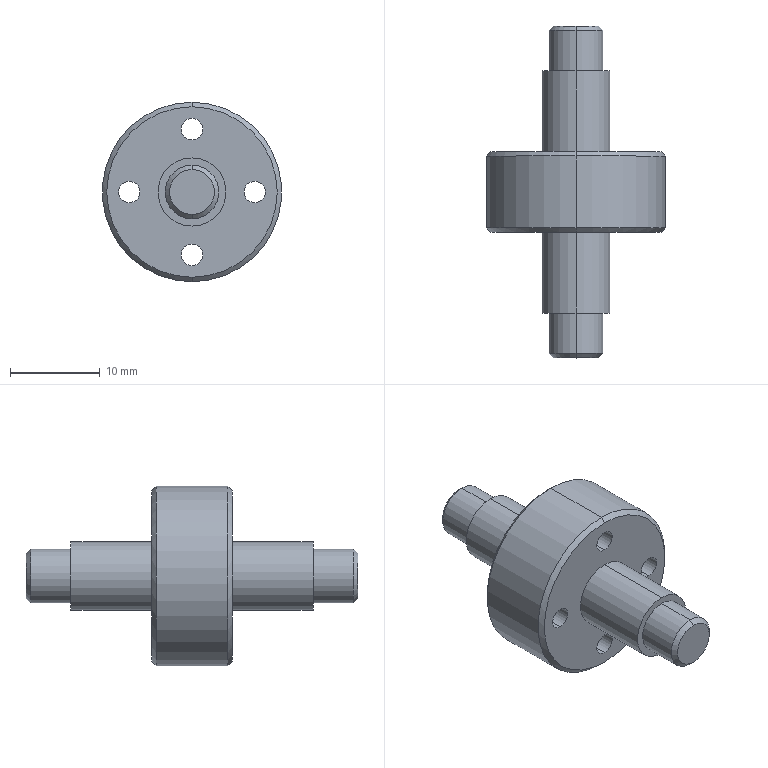Component | SolidWorks | FrontWheelAxis-1 | 1 solid | 32 faces | box 20 x 37 x 20 mm | volume 3744 mm3 | cylinder 18 | cone 8 | plane 6 | commonest cylinder face diameters 2.4 x8 6 x4 7.6 x4 20 x2 | material 6061 Alloy
build123d program:
from build123d import *

# Parameters (mm, degrees)
SKETCH1_R           = 10
SKETCH1_R_2         = 1.2
BOSS_EXTRUDE1_DEPTH = 9
SKETCH2_R           = 3.8
BOSS_EXTRUDE2_DEPTH = 9
SKETCH3_R           = 3
BOSS_EXTRUDE3_DEPTH = 5
BOSS_EXTRUDE4_START = 9
SKETCH4_R           = 3.8
BOSS_EXTRUDE4_DEPTH = 9
BOSS_EXTRUDE5_START = 5
SKETCH5_R           = 3
BOSS_EXTRUDE5_DEPTH = 5
CHAMFER1_SIZE       = 0.5


with BuildPart() as part:
    # Sketch1 → Boss-Extrude1 (new body)
    with BuildSketch(Plane(origin=(0, 0, 0), x_dir=(1, 0, 0), z_dir=(0, 1, 0))):
        with Locations(Location((0, 0, 0), (0, 0, 270))):
            Circle(SKETCH1_R)
        with Locations(Location((7, 0, 0), (0, 0, 270))):
            Circle(SKETCH1_R_2, mode=Mode.SUBTRACT)
        with Locations(Location((0, -7, 0), (0, 0, 270))):
            Circle(SKETCH1_R_2, mode=Mode.SUBTRACT)
        with Locations(Location((-7, 0, 0), (0, 0, 270))):
            Circle(SKETCH1_R_2, mode=Mode.SUBTRACT)
        with Locations(Location((0, 7, 0), (0, 0, 270))):
            Circle(SKETCH1_R_2, mode=Mode.SUBTRACT)
    extrude(amount=BOSS_EXTRUDE1_DEPTH)

    # Sketch2 → Boss-Extrude2 (add)
    with BuildSketch(Plane(origin=(0, 9, 0), x_dir=(1, 0, 0), z_dir=(0, 1, 0))):
        with Locations(Location((0, 0, 0), (0, 0, 270))):
            Circle(SKETCH2_R)
    extrude(amount=BOSS_EXTRUDE2_DEPTH)

    # Sketch3 → Boss-Extrude3 (add)
    with BuildSketch(Plane(origin=(0, 18, 0), x_dir=(1, 0, 0), z_dir=(0, 1, 0))):
        with Locations(Location((0, 0, 0), (0, 0, 270))):
            Circle(SKETCH3_R)
    extrude(amount=BOSS_EXTRUDE3_DEPTH)

    # Sketch4 → Boss-Extrude4 (add)
    with BuildSketch(Plane.XZ.offset(BOSS_EXTRUDE4_START)):
        with Locations(Location((0, 0, 0), (0, 0, 90))):
            Circle(SKETCH4_R)
    extrude(amount=-BOSS_EXTRUDE4_DEPTH)

    # Sketch5 → Boss-Extrude5 (add)
    with BuildSketch(Plane.XZ.offset(9).offset(BOSS_EXTRUDE5_START)):
        with Locations(Location((0, 0, 0), (0, 0, 90))):
            Circle(SKETCH5_R)
    extrude(amount=-BOSS_EXTRUDE5_DEPTH)

    # Chamfer1
    chamfer1_edges = [part.edges().sort_by_distance(p)[0] for p in [
        (0, 0, -10),
        (0, 23, -3),
        (0, -14, -3),
        (0, 9, -10),
    ]]
    chamfer(chamfer1_edges, length=CHAMFER1_SIZE)


solid = part.part

# Placed as in the assembly
solid = solid.moved(Location((0.3183, -0.6003, 37), (0, 0, 0)))
STEP:
#1=CARTESIAN_POINT('',(0.01253,-0.5748,1.358));
#2=VERTEX_POINT('',#1);
#3=CARTESIAN_POINT('',(0.01253,-0.5748,1.555));
#4=VERTEX_POINT('',#3);
#5=CARTESIAN_POINT('',(0.01253,-0.5748,1.457));
#6=DIRECTION('',(0.,-1.,0.));
#7=DIRECTION('',(0.,0.,-1.));
#8=AXIS2_PLACEMENT_3D('',#5,#6,#7);
#9=CIRCLE('',#8,0.09843);
#10=EDGE_CURVE('',#2,#4,#9,.T.);
#11=ORIENTED_EDGE('',*,*,#10,.F.);
#12=CARTESIAN_POINT('',(0.01253,-0.5551,1.339));
#13=VERTEX_POINT('',#12);
#14=CARTESIAN_POINT('',(0.01253,-0.5748,1.358));
#15=DIRECTION('',(0.,0.7071,-0.7071));
#16=VECTOR('',#15,39.37);
#17=LINE('',#14,#16);
#18=EDGE_CURVE('',#2,#13,#17,.T.);
#19=ORIENTED_EDGE('',*,*,#18,.T.);
#20=CARTESIAN_POINT('',(0.01253,-0.5551,1.575));
#21=VERTEX_POINT('',#20);
#22=CARTESIAN_POINT('',(0.01253,-0.5551,1.457));
#23=DIRECTION('',(0.,1.,0.));
#24=DIRECTION('',(0.,0.,-1.));
#25=AXIS2_PLACEMENT_3D('',#22,#23,#24);
#26=CIRCLE('',#25,0.1181);
#27=EDGE_CURVE('',#21,#13,#26,.T.);
#28=ORIENTED_EDGE('',*,*,#27,.F.);
#29=CARTESIAN_POINT('',(0.01253,-0.5748,1.555));
#30=DIRECTION('',(0.,0.7071,0.7071));
#31=VECTOR('',#30,39.37);
#32=LINE('',#29,#31);
#33=EDGE_CURVE('',#4,#21,#32,.T.);
#34=ORIENTED_EDGE('',*,*,#33,.F.);
#35=EDGE_LOOP('',(#11,#19,#28,#34));
#36=FACE_OUTER_BOUND('',#35,.T.);
#37=CARTESIAN_POINT('',(0.01253,-0.5748,1.457));
#38=DIRECTION('',(0.,1.,0.));
#39=DIRECTION('',(0.,0.,1.));
#40=AXIS2_PLACEMENT_3D('',#37,#38,#39);
#41=CONICAL_SURFACE('',#40,0.09843,0.7854);
#42=ADVANCED_FACE('',(#36),#41,.T.);
#43=CARTESIAN_POINT('',(0.01253,0.8819,1.555));
#44=VERTEX_POINT('',#43);
#45=CARTESIAN_POINT('',(0.01253,0.8819,1.358));
#46=VERTEX_POINT('',#45);
#47=CARTESIAN_POINT('',(0.01253,0.8819,1.457));
#48=DIRECTION('',(0.,1.,0.));
#49=DIRECTION('',(0.,0.,1.));
#50=AXIS2_PLACEMENT_3D('',#47,#48,#49);
#51=CIRCLE('',#50,0.09843);
#52=EDGE_CURVE('',#44,#46,#51,.T.);
#53=ORIENTED_EDGE('',*,*,#52,.F.);
#54=CARTESIAN_POINT('',(0.01253,0.8622,1.575));
#55=VERTEX_POINT('',#54);
#56=CARTESIAN_POINT('',(0.01253,0.8819,1.555));
#57=DIRECTION('',(0.,-0.7071,0.7071));
#58=VECTOR('',#57,39.37);
#59=LINE('',#56,#58);
#60=EDGE_CURVE('',#44,#55,#59,.T.);
#61=ORIENTED_EDGE('',*,*,#60,.T.);
#62=CARTESIAN_POINT('',(0.01253,0.8622,1.339));
#63=VERTEX_POINT('',#62);
#64=CARTESIAN_POINT('',(0.01253,0.8622,1.457));
#65=DIRECTION('',(0.,-1.,0.));
#66=DIRECTION('',(0.,0.,1.));
#67=AXIS2_PLACEMENT_3D('',#64,#65,#66);
#68=CIRCLE('',#67,0.1181);
#69=EDGE_CURVE('',#63,#55,#68,.T.);
#70=ORIENTED_EDGE('',*,*,#69,.F.);
#71=CARTESIAN_POINT('',(0.01253,0.8819,1.358));
#72=DIRECTION('',(0.,-0.7071,-0.7071));
#73=VECTOR('',#72,39.37);
#74=LINE('',#71,#73);
#75=EDGE_CURVE('',#46,#63,#74,.T.);
#76=ORIENTED_EDGE('',*,*,#75,.F.);
#77=EDGE_LOOP('',(#53,#61,#70,#76));
#78=FACE_OUTER_BOUND('',#77,.T.);
#79=CARTESIAN_POINT('',(0.01253,0.8819,1.457));
#80=DIRECTION('',(0.,-1.,0.));
#81=DIRECTION('',(0.,0.,-1.));
#82=AXIS2_PLACEMENT_3D('',#79,#80,#81);
#83=CONICAL_SURFACE('',#82,0.09843,0.7854);
#84=ADVANCED_FACE('',(#78),#83,.T.);
#85=CARTESIAN_POINT('',(0.01253,-0.02363,1.083));
#86=VERTEX_POINT('',#85);
#87=CARTESIAN_POINT('',(0.01253,-0.02363,1.831));
#88=VERTEX_POINT('',#87);
#89=CARTESIAN_POINT('',(0.01253,-0.02363,1.457));
#90=DIRECTION('',(0.,-1.,0.));
#91=DIRECTION('',(0.,0.,1.));
#92=AXIS2_PLACEMENT_3D('',#89,#90,#91);
#93=CIRCLE('',#92,0.374);
#94=EDGE_CURVE('',#86,#88,#93,.T.);
#95=ORIENTED_EDGE('',*,*,#94,.F.);
#96=CARTESIAN_POINT('',(0.01253,-0.003948,1.063));
#97=VERTEX_POINT('',#96);
#98=CARTESIAN_POINT('',(0.01253,-0.003948,1.063));
#99=DIRECTION('',(0.,0.7071,-0.7071));
#100=VECTOR('',#99,39.37);
#101=LINE('',#98,#100);
#102=EDGE_CURVE('',#86,#97,#101,.T.);
#103=ORIENTED_EDGE('',*,*,#102,.T.);
#104=CARTESIAN_POINT('',(0.01253,-0.003948,1.85));
#105=VERTEX_POINT('',#104);
#106=CARTESIAN_POINT('',(0.01253,-0.003948,1.457));
#107=DIRECTION('',(0.,1.,0.));
#108=DIRECTION('',(0.,0.,1.));
#109=AXIS2_PLACEMENT_3D('',#106,#107,#108);
#110=CIRCLE('',#109,0.3937);
#111=EDGE_CURVE('',#105,#97,#110,.T.);
#112=ORIENTED_EDGE('',*,*,#111,.F.);
#113=CARTESIAN_POINT('',(0.01253,-0.003948,1.85));
#114=DIRECTION('',(0.,0.7071,0.7071));
#115=VECTOR('',#114,39.37);
#116=LINE('',#113,#115);
#117=EDGE_CURVE('',#88,#105,#116,.T.);
#118=ORIENTED_EDGE('',*,*,#117,.F.);
#119=EDGE_LOOP('',(#95,#103,#112,#118));
#120=FACE_OUTER_BOUND('',#119,.T.);
#121=CARTESIAN_POINT('',(0.01253,-0.003948,1.457));
#122=DIRECTION('',(0.,1.,0.));
#123=DIRECTION('',(0.,0.,1.));
#124=AXIS2_PLACEMENT_3D('',#121,#122,#123);
#125=CONICAL_SURFACE('',#124,0.3937,0.7854);
#126=ADVANCED_FACE('',(#120),#125,.T.);
#127=CARTESIAN_POINT('',(0.01253,0.3307,1.831));
#128=VERTEX_POINT('',#127);
#129=CARTESIAN_POINT('',(0.01253,0.3307,1.083));
#130=VERTEX_POINT('',#129);
#131=CARTESIAN_POINT('',(0.01253,0.3307,1.457));
#132=DIRECTION('',(0.,1.,0.));
#133=DIRECTION('',(0.,0.,1.));
#134=AXIS2_PLACEMENT_3D('',#131,#132,#133);
#135=CIRCLE('',#134,0.374);
#136=EDGE_CURVE('',#128,#130,#135,.T.);
#137=ORIENTED_EDGE('',*,*,#136,.F.);
#138=CARTESIAN_POINT('',(0.01253,0.311,1.85));
#139=VERTEX_POINT('',#138);
#140=CARTESIAN_POINT('',(0.01253,0.3307,1.831));
#141=DIRECTION('',(0.,-0.7071,0.7071));
#142=VECTOR('',#141,39.37);
#143=LINE('',#140,#142);
#144=EDGE_CURVE('',#128,#139,#143,.T.);
#145=ORIENTED_EDGE('',*,*,#144,.T.);
#146=CARTESIAN_POINT('',(0.01253,0.311,1.063));
#147=VERTEX_POINT('',#146);
#148=CARTESIAN_POINT('',(0.01253,0.311,1.457));
#149=DIRECTION('',(0.,-1.,0.));
#150=DIRECTION('',(0.,0.,1.));
#151=AXIS2_PLACEMENT_3D('',#148,#149,#150);
#152=CIRCLE('',#151,0.3937);
#153=EDGE_CURVE('',#147,#139,#152,.T.);
#154=ORIENTED_EDGE('',*,*,#153,.F.);
#155=CARTESIAN_POINT('',(0.01253,0.3307,1.083));
#156=DIRECTION('',(0.,-0.7071,-0.7071));
#157=VECTOR('',#156,39.37);
#158=LINE('',#155,#157);
#159=EDGE_CURVE('',#130,#147,#158,.T.);
#160=ORIENTED_EDGE('',*,*,#159,.F.);
#161=EDGE_LOOP('',(#137,#145,#154,#160));
#162=FACE_OUTER_BOUND('',#161,.T.);
#163=CARTESIAN_POINT('',(0.01253,0.3307,1.457));
#164=DIRECTION('',(0.,-1.,0.));
#165=DIRECTION('',(0.,0.,-1.));
#166=AXIS2_PLACEMENT_3D('',#163,#164,#165);
#167=CONICAL_SURFACE('',#166,0.374,0.7854);
#168=ADVANCED_FACE('',(#162),#167,.T.);
#169=ORIENTED_EDGE('',*,*,#27,.T.);
#170=CARTESIAN_POINT('',(0.01253,-0.378,1.339));
#171=VERTEX_POINT('',#170);
#172=CARTESIAN_POINT('',(0.01253,-0.5748,1.339));
#173=DIRECTION('',(0.,1.,0.));
#174=VECTOR('',#173,39.37);
#175=LINE('',#172,#174);
#176=EDGE_CURVE('',#13,#171,#175,.T.);
#177=ORIENTED_EDGE('',*,*,#176,.T.);
#178=CARTESIAN_POINT('',(0.01253,-0.378,1.575));
#179=VERTEX_POINT('',#178);
#180=CARTESIAN_POINT('',(0.01253,-0.378,1.457));
#181=DIRECTION('',(0.,-1.,0.));
#182=DIRECTION('',(0.,0.,-1.));
#183=AXIS2_PLACEMENT_3D('',#180,#181,#182);
#184=CIRCLE('',#183,0.1181);
#185=EDGE_CURVE('',#171,#179,#184,.T.);
#186=ORIENTED_EDGE('',*,*,#185,.T.);
#187=CARTESIAN_POINT('',(0.01253,-0.5748,1.575));
#188=DIRECTION('',(0.,1.,0.));
#189=VECTOR('',#188,39.37);
#190=LINE('',#187,#189);
#191=EDGE_CURVE('',#21,#179,#190,.T.);
#192=ORIENTED_EDGE('',*,*,#191,.F.);
#193=EDGE_LOOP('',(#169,#177,#186,#192));
#194=FACE_OUTER_BOUND('',#193,.T.);
#195=CARTESIAN_POINT('',(0.01253,-0.5748,1.457));
#196=DIRECTION('',(0.,1.,0.));
#197=DIRECTION('',(0.,0.,1.));
#198=AXIS2_PLACEMENT_3D('',#195,#196,#197);
#199=CYLINDRICAL_SURFACE('',#198,0.1181);
#200=ADVANCED_FACE('',(#194),#199,.T.);
#201=CARTESIAN_POINT('',(0.01253,-0.378,1.307));
#202=VERTEX_POINT('',#201);
#203=CARTESIAN_POINT('',(0.01253,-0.378,1.606));
#204=VERTEX_POINT('',#203);
#205=CARTESIAN_POINT('',(0.01253,-0.378,1.457));
#206=DIRECTION('',(0.,-1.,0.));
#207=DIRECTION('',(0.,0.,-1.));
#208=AXIS2_PLACEMENT_3D('',#205,#206,#207);
#209=CIRCLE('',#208,0.1496);
#210=EDGE_CURVE('',#202,#204,#209,.T.);
#211=ORIENTED_EDGE('',*,*,#210,.F.);
#212=CARTESIAN_POINT('',(0.01253,-0.02363,1.307));
#213=VERTEX_POINT('',#212);
#214=CARTESIAN_POINT('',(0.01253,-0.378,1.307));
#215=DIRECTION('',(0.,1.,0.));
#216=VECTOR('',#215,39.37);
#217=LINE('',#214,#216);
#218=EDGE_CURVE('',#202,#213,#217,.T.);
#219=ORIENTED_EDGE('',*,*,#218,.T.);
#220=CARTESIAN_POINT('',(0.01253,-0.02363,1.606));
#221=VERTEX_POINT('',#220);
#222=CARTESIAN_POINT('',(0.01253,-0.02363,1.457));
#223=DIRECTION('',(0.,-1.,0.));
#224=DIRECTION('',(0.,0.,1.));
#225=AXIS2_PLACEMENT_3D('',#222,#223,#224);
#226=CIRCLE('',#225,0.1496);
#227=EDGE_CURVE('',#213,#221,#226,.T.);
#228=ORIENTED_EDGE('',*,*,#227,.T.);
#229=CARTESIAN_POINT('',(0.01253,-0.378,1.606));
#230=DIRECTION('',(0.,1.,0.));
#231=VECTOR('',#230,39.37);
#232=LINE('',#229,#231);
#233=EDGE_CURVE('',#204,#221,#232,.T.);
#234=ORIENTED_EDGE('',*,*,#233,.F.);
#235=EDGE_LOOP('',(#211,#219,#228,#234));
#236=FACE_OUTER_BOUND('',#235,.T.);
#237=CARTESIAN_POINT('',(0.01253,-0.378,1.457));
#238=DIRECTION('',(0.,1.,0.));
#239=DIRECTION('',(0.,0.,1.));
#240=AXIS2_PLACEMENT_3D('',#237,#238,#239);
#241=CYLINDRICAL_SURFACE('',#240,0.1496);
#242=ADVANCED_FACE('',(#236),#241,.T.);
#243=ORIENTED_EDGE('',*,*,#69,.T.);
#244=CARTESIAN_POINT('',(0.01253,0.685,1.575));
#245=VERTEX_POINT('',#244);
#246=CARTESIAN_POINT('',(0.01253,0.8819,1.575));
#247=DIRECTION('',(0.,-1.,0.));
#248=VECTOR('',#247,39.37);
#249=LINE('',#246,#248);
#250=EDGE_CURVE('',#55,#245,#249,.T.);
#251=ORIENTED_EDGE('',*,*,#250,.T.);
#252=CARTESIAN_POINT('',(0.01253,0.685,1.339));
#253=VERTEX_POINT('',#252);
#254=CARTESIAN_POINT('',(0.01253,0.685,1.457));
#255=DIRECTION('',(0.,1.,0.));
#256=DIRECTION('',(0.,0.,1.));
#257=AXIS2_PLACEMENT_3D('',#254,#255,#256);
#258=CIRCLE('',#257,0.1181);
#259=EDGE_CURVE('',#245,#253,#258,.T.);
#260=ORIENTED_EDGE('',*,*,#259,.T.);
#261=CARTESIAN_POINT('',(0.01253,0.8819,1.339));
#262=DIRECTION('',(0.,-1.,0.));
#263=VECTOR('',#262,39.37);
#264=LINE('',#261,#263);
#265=EDGE_CURVE('',#63,#253,#264,.T.);
#266=ORIENTED_EDGE('',*,*,#265,.F.);
#267=EDGE_LOOP('',(#243,#251,#260,#266));
#268=FACE_OUTER_BOUND('',#267,.T.);
#269=CARTESIAN_POINT('',(0.01253,0.8819,1.457));
#270=DIRECTION('',(0.,-1.,0.));
#271=DIRECTION('',(0.,0.,-1.));
#272=AXIS2_PLACEMENT_3D('',#269,#270,#271);
#273=CYLINDRICAL_SURFACE('',#272,0.1181);
#274=ADVANCED_FACE('',(#268),#273,.T.);
#275=CARTESIAN_POINT('',(0.01253,0.685,1.606));
#276=VERTEX_POINT('',#275);
#277=CARTESIAN_POINT('',(0.01253,0.685,1.307));
#278=VERTEX_POINT('',#277);
#279=CARTESIAN_POINT('',(0.01253,0.685,1.457));
#280=DIRECTION('',(0.,1.,0.));
#281=DIRECTION('',(0.,0.,1.));
#282=AXIS2_PLACEMENT_3D('',#279,#280,#281);
#283=CIRCLE('',#282,0.1496);
#284=EDGE_CURVE('',#276,#278,#283,.T.);
#285=ORIENTED_EDGE('',*,*,#284,.F.);
#286=CARTESIAN_POINT('',(0.01253,0.3307,1.606));
#287=VERTEX_POINT('',#286);
#288=CARTESIAN_POINT('',(0.01253,0.685,1.606));
#289=DIRECTION('',(0.,-1.,0.));
#290=VECTOR('',#289,39.37);
#291=LINE('',#288,#290);
#292=EDGE_CURVE('',#276,#287,#291,.T.);
#293=ORIENTED_EDGE('',*,*,#292,.T.);
#294=CARTESIAN_POINT('',(0.01253,0.3307,1.307));
#295=VERTEX_POINT('',#294);
#296=CARTESIAN_POINT('',(0.01253,0.3307,1.457));
#297=DIRECTION('',(0.,1.,0.));
#298=DIRECTION('',(0.,0.,1.));
#299=AXIS2_PLACEMENT_3D('',#296,#297,#298);
#300=CIRCLE('',#299,0.1496);
#301=EDGE_CURVE('',#287,#295,#300,.T.);
#302=ORIENTED_EDGE('',*,*,#301,.T.);
#303=CARTESIAN_POINT('',(0.01253,0.685,1.307));
#304=DIRECTION('',(0.,-1.,0.));
#305=VECTOR('',#304,39.37);
#306=LINE('',#303,#305);
#307=EDGE_CURVE('',#278,#295,#306,.T.);
#308=ORIENTED_EDGE('',*,*,#307,.F.);
#309=EDGE_LOOP('',(#285,#293,#302,#308));
#310=FACE_OUTER_BOUND('',#309,.T.);
#311=CARTESIAN_POINT('',(0.01253,0.685,1.457));
#312=DIRECTION('',(0.,-1.,0.));
#313=DIRECTION('',(0.,0.,-1.));
#314=AXIS2_PLACEMENT_3D('',#311,#312,#313);
#315=CYLINDRICAL_SURFACE('',#314,0.1496);
#316=ADVANCED_FACE('',(#310),#315,.T.);
#317=CARTESIAN_POINT('',(0.01253,0.3307,1.134));
#318=VERTEX_POINT('',#317);
#319=CARTESIAN_POINT('',(0.01253,0.3307,1.228));
#320=VERTEX_POINT('',#319);
#321=CARTESIAN_POINT('',(0.01253,0.3307,1.181));
#322=DIRECTION('',(0.,1.,0.));
#323=DIRECTION('',(0.,0.,1.));
#324=AXIS2_PLACEMENT_3D('',#321,#322,#323);
#325=CIRCLE('',#324,0.04724);
#326=EDGE_CURVE('',#318,#320,#325,.T.);
#327=ORIENTED_EDGE('',*,*,#326,.T.);
#328=CARTESIAN_POINT('',(0.01253,-0.02363,1.228));
#329=VERTEX_POINT('',#328);
#330=CARTESIAN_POINT('',(0.01253,0.3307,1.228));
#331=DIRECTION('',(0.,-1.,0.));
#332=VECTOR('',#331,39.37);
#333=LINE('',#330,#332);
#334=EDGE_CURVE('',#320,#329,#333,.T.);
#335=ORIENTED_EDGE('',*,*,#334,.T.);
#336=CARTESIAN_POINT('',(0.01253,-0.02363,1.134));
#337=VERTEX_POINT('',#336);
#338=CARTESIAN_POINT('',(0.01253,-0.02363,1.181));
#339=DIRECTION('',(0.,1.,0.));
#340=DIRECTION('',(0.,0.,1.));
#341=AXIS2_PLACEMENT_3D('',#338,#339,#340);
#342=CIRCLE('',#341,0.04724);
#343=EDGE_CURVE('',#337,#329,#342,.T.);
#344=ORIENTED_EDGE('',*,*,#343,.F.);
#345=CARTESIAN_POINT('',(0.01253,0.3307,1.134));
#346=DIRECTION('',(0.,-1.,0.));
#347=VECTOR('',#346,39.37);
#348=LINE('',#345,#347);
#349=EDGE_CURVE('',#318,#337,#348,.T.);
#350=ORIENTED_EDGE('',*,*,#349,.F.);
#351=EDGE_LOOP('',(#327,#335,#344,#350));
#352=FACE_OUTER_BOUND('',#351,.T.);
#353=CARTESIAN_POINT('',(0.01253,0.3307,1.181));
#354=DIRECTION('',(0.,-1.,0.));
#355=DIRECTION('',(0.,0.,-1.));
#356=AXIS2_PLACEMENT_3D('',#353,#354,#355);
#357=CYLINDRICAL_SURFACE('',#356,0.04724);
#358=ADVANCED_FACE('',(#352),#357,.F.);
#359=CARTESIAN_POINT('',(-0.2631,0.3307,1.409));
#360=VERTEX_POINT('',#359);
#361=CARTESIAN_POINT('',(-0.2631,0.3307,1.504));
#362=VERTEX_POINT('',#361);
#363=CARTESIAN_POINT('',(-0.2631,0.3307,1.457));
#364=DIRECTION('',(0.,1.,0.));
#365=DIRECTION('',(0.,0.,1.));
#366=AXIS2_PLACEMENT_3D('',#363,#364,#365);
#367=CIRCLE('',#366,0.04724);
#368=EDGE_CURVE('',#360,#362,#367,.T.);
#369=ORIENTED_EDGE('',*,*,#368,.T.);
#370=CARTESIAN_POINT('',(-0.2631,-0.02363,1.504));
#371=VERTEX_POINT('',#370);
#372=CARTESIAN_POINT('',(-0.2631,0.3307,1.504));
#373=DIRECTION('',(0.,-1.,0.));
#374=VECTOR('',#373,39.37);
#375=LINE('',#372,#374);
#376=EDGE_CURVE('',#362,#371,#375,.T.);
#377=ORIENTED_EDGE('',*,*,#376,.T.);
#378=CARTESIAN_POINT('',(-0.2631,-0.02363,1.409));
#379=VERTEX_POINT('',#378);
#380=CARTESIAN_POINT('',(-0.2631,-0.02363,1.457));
#381=DIRECTION('',(0.,1.,0.));
#382=DIRECTION('',(0.,0.,1.));
#383=AXIS2_PLACEMENT_3D('',#380,#381,#382);
#384=CIRCLE('',#383,0.04724);
#385=EDGE_CURVE('',#379,#371,#384,.T.);
#386=ORIENTED_EDGE('',*,*,#385,.F.);
#387=CARTESIAN_POINT('',(-0.2631,0.3307,1.409));
#388=DIRECTION('',(0.,-1.,0.));
#389=VECTOR('',#388,39.37);
#390=LINE('',#387,#389);
#391=EDGE_CURVE('',#360,#379,#390,.T.);
#392=ORIENTED_EDGE('',*,*,#391,.F.);
#393=EDGE_LOOP('',(#369,#377,#386,#392));
#394=FACE_OUTER_BOUND('',#393,.T.);
#395=CARTESIAN_POINT('',(-0.2631,0.3307,1.457));
#396=DIRECTION('',(0.,-1.,0.));
#397=DIRECTION('',(0.,0.,-1.));
#398=AXIS2_PLACEMENT_3D('',#395,#396,#397);
#399=CYLINDRICAL_SURFACE('',#398,0.04724);
#400=ADVANCED_FACE('',(#394),#399,.F.);
#401=CARTESIAN_POINT('',(0.01253,0.3307,1.685));
#402=VERTEX_POINT('',#401);
#403=CARTESIAN_POINT('',(0.01253,0.3307,1.78));
#404=VERTEX_POINT('',#403);
#405=CARTESIAN_POINT('',(0.01253,0.3307,1.732));
#406=DIRECTION('',(0.,1.,0.));
#407=DIRECTION('',(0.,0.,1.));
#408=AXIS2_PLACEMENT_3D('',#405,#406,#407);
#409=CIRCLE('',#408,0.04724);
#410=EDGE_CURVE('',#402,#404,#409,.T.);
#411=ORIENTED_EDGE('',*,*,#410,.T.);
#412=CARTESIAN_POINT('',(0.01253,-0.02363,1.78));
#413=VERTEX_POINT('',#412);
#414=CARTESIAN_POINT('',(0.01253,0.3307,1.78));
#415=DIRECTION('',(0.,-1.,0.));
#416=VECTOR('',#415,39.37);
#417=LINE('',#414,#416);
#418=EDGE_CURVE('',#404,#413,#417,.T.);
#419=ORIENTED_EDGE('',*,*,#418,.T.);
#420=CARTESIAN_POINT('',(0.01253,-0.02363,1.685));
#421=VERTEX_POINT('',#420);
#422=CARTESIAN_POINT('',(0.01253,-0.02363,1.732));
#423=DIRECTION('',(0.,1.,0.));
#424=DIRECTION('',(0.,0.,1.));
#425=AXIS2_PLACEMENT_3D('',#422,#423,#424);
#426=CIRCLE('',#425,0.04724);
#427=EDGE_CURVE('',#421,#413,#426,.T.);
#428=ORIENTED_EDGE('',*,*,#427,.F.);
#429=CARTESIAN_POINT('',(0.01253,0.3307,1.685));
#430=DIRECTION('',(0.,-1.,0.));
#431=VECTOR('',#430,39.37);
#432=LINE('',#429,#431);
#433=EDGE_CURVE('',#402,#421,#432,.T.);
#434=ORIENTED_EDGE('',*,*,#433,.F.);
#435=EDGE_LOOP('',(#411,#419,#428,#434));
#436=FACE_OUTER_BOUND('',#435,.T.);
#437=CARTESIAN_POINT('',(0.01253,0.3307,1.732));
#438=DIRECTION('',(0.,-1.,0.));
#439=DIRECTION('',(0.,0.,-1.));
#440=AXIS2_PLACEMENT_3D('',#437,#438,#439);
#441=CYLINDRICAL_SURFACE('',#440,0.04724);
#442=ADVANCED_FACE('',(#436),#441,.F.);
#443=CARTESIAN_POINT('',(0.2881,0.3307,1.409));
#444=VERTEX_POINT('',#443);
#445=CARTESIAN_POINT('',(0.2881,0.3307,1.504));
#446=VERTEX_POINT('',#445);
#447=CARTESIAN_POINT('',(0.2881,0.3307,1.457));
#448=DIRECTION('',(0.,1.,0.));
#449=DIRECTION('',(0.,0.,1.));
#450=AXIS2_PLACEMENT_3D('',#447,#448,#449);
#451=CIRCLE('',#450,0.04724);
#452=EDGE_CURVE('',#444,#446,#451,.T.);
#453=ORIENTED_EDGE('',*,*,#452,.T.);
#454=CARTESIAN_POINT('',(0.2881,-0.02363,1.504));
#455=VERTEX_POINT('',#454);
#456=CARTESIAN_POINT('',(0.2881,0.3307,1.504));
#457=DIRECTION('',(0.,-1.,0.));
#458=VECTOR('',#457,39.37);
#459=LINE('',#456,#458);
#460=EDGE_CURVE('',#446,#455,#459,.T.);
#461=ORIENTED_EDGE('',*,*,#460,.T.);
#462=CARTESIAN_POINT('',(0.2881,-0.02363,1.409));
#463=VERTEX_POINT('',#462);
#464=CARTESIAN_POINT('',(0.2881,-0.02363,1.457));
#465=DIRECTION('',(0.,1.,0.));
#466=DIRECTION('',(0.,0.,1.));
#467=AXIS2_PLACEMENT_3D('',#464,#465,#466);
#468=CIRCLE('',#467,0.04724);
#469=EDGE_CURVE('',#463,#455,#468,.T.);
#470=ORIENTED_EDGE('',*,*,#469,.F.);
#471=CARTESIAN_POINT('',(0.2881,0.3307,1.409));
#472=DIRECTION('',(0.,-1.,0.));
#473=VECTOR('',#472,39.37);
#474=LINE('',#471,#473);
#475=EDGE_CURVE('',#444,#463,#474,.T.);
#476=ORIENTED_EDGE('',*,*,#475,.F.);
#477=EDGE_LOOP('',(#453,#461,#470,#476));
#478=FACE_OUTER_BOUND('',#477,.T.);
#479=CARTESIAN_POINT('',(0.2881,0.3307,1.457));
#480=DIRECTION('',(0.,-1.,0.));
#481=DIRECTION('',(0.,0.,-1.));
#482=AXIS2_PLACEMENT_3D('',#479,#480,#481);
#483=CYLINDRICAL_SURFACE('',#482,0.04724);
#484=ADVANCED_FACE('',(#478),#483,.F.);
#485=ORIENTED_EDGE('',*,*,#153,.T.);
#486=CARTESIAN_POINT('',(0.01253,0.3307,1.85));
#487=DIRECTION('',(0.,-1.,0.));
#488=VECTOR('',#487,39.37);
#489=LINE('',#486,#488);
#490=EDGE_CURVE('',#139,#105,#489,.T.);
#491=ORIENTED_EDGE('',*,*,#490,.T.);
#492=ORIENTED_EDGE('',*,*,#111,.T.);
#493=CARTESIAN_POINT('',(0.01253,0.3307,1.063));
#494=DIRECTION('',(0.,-1.,0.));
#495=VECTOR('',#494,39.37);
#496=LINE('',#493,#495);
#497=EDGE_CURVE('',#147,#97,#496,.T.);
#498=ORIENTED_EDGE('',*,*,#497,.F.);
#499=EDGE_LOOP('',(#485,#491,#492,#498));
#500=FACE_OUTER_BOUND('',#499,.T.);
#501=CARTESIAN_POINT('',(0.01253,0.3307,1.457));
#502=DIRECTION('',(0.,-1.,0.));
#503=DIRECTION('',(0.,0.,-1.));
#504=AXIS2_PLACEMENT_3D('',#501,#502,#503);
#505=CYLINDRICAL_SURFACE('',#504,0.3937);
#506=ADVANCED_FACE('',(#500),#505,.T.);
#507=CARTESIAN_POINT('',(0.01253,-0.378,1.457));
#508=DIRECTION('',(0.,-1.,0.));
#509=DIRECTION('',(0.,0.,-1.));
#510=AXIS2_PLACEMENT_3D('',#507,#508,#509);
#511=CIRCLE('',#510,0.1496);
#512=EDGE_CURVE('',#204,#202,#511,.T.);
#513=ORIENTED_EDGE('',*,*,#512,.T.);
#514=ORIENTED_EDGE('',*,*,#210,.T.);
#515=EDGE_LOOP('',(#513,#514));
#516=FACE_OUTER_BOUND('',#515,.T.);
#517=CARTESIAN_POINT('',(0.01253,-0.378,1.457));
#518=DIRECTION('',(0.,-1.,0.));
#519=DIRECTION('',(0.,0.,-1.));
#520=AXIS2_PLACEMENT_3D('',#517,#518,#519);
#521=CIRCLE('',#520,0.1181);
#522=EDGE_CURVE('',#179,#171,#521,.T.);
#523=ORIENTED_EDGE('',*,*,#522,.F.);
#524=ORIENTED_EDGE('',*,*,#185,.F.);
#525=EDGE_LOOP('',(#523,#524));
#526=FACE_BOUND('',#525,.T.);
#527=CARTESIAN_POINT('',(0.01253,-0.378,1.457));
#528=DIRECTION('',(0.,-1.,0.));
#529=DIRECTION('',(0.,0.,-1.));
#530=AXIS2_PLACEMENT_3D('',#527,#528,#529);
#531=PLANE('',#530);
#532=ADVANCED_FACE('',(#516,#526),#531,.T.);
#533=CARTESIAN_POINT('',(0.01253,-0.02363,1.457));
#534=DIRECTION('',(0.,-1.,0.));
#535=DIRECTION('',(0.,0.,1.));
#536=AXIS2_PLACEMENT_3D('',#533,#534,#535);
#537=CIRCLE('',#536,0.374);
#538=EDGE_CURVE('',#88,#86,#537,.T.);
#539=ORIENTED_EDGE('',*,*,#538,.T.);
#540=ORIENTED_EDGE('',*,*,#94,.T.);
#541=EDGE_LOOP('',(#539,#540));
#542=FACE_OUTER_BOUND('',#541,.T.);
#543=ORIENTED_EDGE('',*,*,#469,.T.);
#544=CARTESIAN_POINT('',(0.2881,-0.02363,1.457));
#545=DIRECTION('',(0.,1.,0.));
#546=DIRECTION('',(0.,0.,1.));
#547=AXIS2_PLACEMENT_3D('',#544,#545,#546);
#548=CIRCLE('',#547,0.04724);
#549=EDGE_CURVE('',#455,#463,#548,.T.);
#550=ORIENTED_EDGE('',*,*,#549,.T.);
#551=EDGE_LOOP('',(#543,#550));
#552=FACE_BOUND('',#551,.T.);
#553=ORIENTED_EDGE('',*,*,#427,.T.);
#554=CARTESIAN_POINT('',(0.01253,-0.02363,1.732));
#555=DIRECTION('',(0.,1.,0.));
#556=DIRECTION('',(0.,0.,1.));
#557=AXIS2_PLACEMENT_3D('',#554,#555,#556);
#558=CIRCLE('',#557,0.04724);
#559=EDGE_CURVE('',#413,#421,#558,.T.);
#560=ORIENTED_EDGE('',*,*,#559,.T.);
#561=EDGE_LOOP('',(#553,#560));
#562=FACE_BOUND('',#561,.T.);
#563=ORIENTED_EDGE('',*,*,#385,.T.);
#564=CARTESIAN_POINT('',(-0.2631,-0.02363,1.457));
#565=DIRECTION('',(0.,1.,0.));
#566=DIRECTION('',(0.,0.,1.));
#567=AXIS2_PLACEMENT_3D('',#564,#565,#566);
#568=CIRCLE('',#567,0.04724);
#569=EDGE_CURVE('',#371,#379,#568,.T.);
#570=ORIENTED_EDGE('',*,*,#569,.T.);
#571=EDGE_LOOP('',(#563,#570));
#572=FACE_BOUND('',#571,.T.);
#573=ORIENTED_EDGE('',*,*,#343,.T.);
#574=CARTESIAN_POINT('',(0.01253,-0.02363,1.181));
#575=DIRECTION('',(0.,1.,0.));
#576=DIRECTION('',(0.,0.,1.));
#577=AXIS2_PLACEMENT_3D('',#574,#575,#576);
#578=CIRCLE('',#577,0.04724);
#579=EDGE_CURVE('',#329,#337,#578,.T.);
#580=ORIENTED_EDGE('',*,*,#579,.T.);
#581=EDGE_LOOP('',(#573,#580));
#582=FACE_BOUND('',#581,.T.);
#583=CARTESIAN_POINT('',(0.01253,-0.02363,1.457));
#584=DIRECTION('',(0.,-1.,0.));
#585=DIRECTION('',(0.,0.,1.));
#586=AXIS2_PLACEMENT_3D('',#583,#584,#585);
#587=CIRCLE('',#586,0.1496);
#588=EDGE_CURVE('',#221,#213,#587,.T.);
#589=ORIENTED_EDGE('',*,*,#588,.F.);
#590=ORIENTED_EDGE('',*,*,#227,.F.);
#591=EDGE_LOOP('',(#589,#590));
#592=FACE_BOUND('',#591,.T.);
#593=CARTESIAN_POINT('',(0.01253,-0.02363,1.457));
#594=DIRECTION('',(0.,1.,0.));
#595=DIRECTION('',(0.,0.,1.));
#596=AXIS2_PLACEMENT_3D('',#593,#594,#595);
#597=PLANE('',#596);
#598=ADVANCED_FACE('',(#542,#552,#562,#572,#582,#592),#597,.F.);
#599=CARTESIAN_POINT('',(0.01253,0.685,1.457));
#600=DIRECTION('',(0.,1.,0.));
#601=DIRECTION('',(0.,0.,1.));
#602=AXIS2_PLACEMENT_3D('',#599,#600,#601);
#603=CIRCLE('',#602,0.1496);
#604=EDGE_CURVE('',#278,#276,#603,.T.);
#605=ORIENTED_EDGE('',*,*,#604,.T.);
#606=ORIENTED_EDGE('',*,*,#284,.T.);
#607=EDGE_LOOP('',(#605,#606));
#608=FACE_OUTER_BOUND('',#607,.T.);
#609=CARTESIAN_POINT('',(0.01253,0.685,1.457));
#610=DIRECTION('',(0.,1.,0.));
#611=DIRECTION('',(0.,0.,1.));
#612=AXIS2_PLACEMENT_3D('',#609,#610,#611);
#613=CIRCLE('',#612,0.1181);
#614=EDGE_CURVE('',#253,#245,#613,.T.);
#615=ORIENTED_EDGE('',*,*,#614,.F.);
#616=ORIENTED_EDGE('',*,*,#259,.F.);
#617=EDGE_LOOP('',(#615,#616));
#618=FACE_BOUND('',#617,.T.);
#619=CARTESIAN_POINT('',(0.01253,0.685,1.457));
#620=DIRECTION('',(0.,1.,0.));
#621=DIRECTION('',(0.,0.,1.));
#622=AXIS2_PLACEMENT_3D('',#619,#620,#621);
#623=PLANE('',#622);
#624=ADVANCED_FACE('',(#608,#618),#623,.T.);
#625=CARTESIAN_POINT('',(0.01253,0.3307,1.457));
#626=DIRECTION('',(0.,1.,0.));
#627=DIRECTION('',(0.,0.,1.));
#628=AXIS2_PLACEMENT_3D('',#625,#626,#627);
#629=CIRCLE('',#628,0.374);
#630=EDGE_CURVE('',#130,#128,#629,.T.);
#631=ORIENTED_EDGE('',*,*,#630,.T.);
#632=ORIENTED_EDGE('',*,*,#136,.T.);
#633=EDGE_LOOP('',(#631,#632));
#634=FACE_OUTER_BOUND('',#633,.T.);
#635=ORIENTED_EDGE('',*,*,#326,.F.);
#636=CARTESIAN_POINT('',(0.01253,0.3307,1.181));
#637=DIRECTION('',(0.,1.,0.));
#638=DIRECTION('',(0.,0.,1.));
#639=AXIS2_PLACEMENT_3D('',#636,#637,#638);
#640=CIRCLE('',#639,0.04724);
#641=EDGE_CURVE('',#320,#318,#640,.T.);
#642=ORIENTED_EDGE('',*,*,#641,.F.);
#643=EDGE_LOOP('',(#635,#642));
#644=FACE_BOUND('',#643,.T.);
#645=ORIENTED_EDGE('',*,*,#410,.F.);
#646=CARTESIAN_POINT('',(0.01253,0.3307,1.732));
#647=DIRECTION('',(0.,1.,0.));
#648=DIRECTION('',(0.,0.,1.));
#649=AXIS2_PLACEMENT_3D('',#646,#647,#648);
#650=CIRCLE('',#649,0.04724);
#651=EDGE_CURVE('',#404,#402,#650,.T.);
#652=ORIENTED_EDGE('',*,*,#651,.F.);
#653=EDGE_LOOP('',(#645,#652));
#654=FACE_BOUND('',#653,.T.);
#655=ORIENTED_EDGE('',*,*,#452,.F.);
#656=CARTESIAN_POINT('',(0.2881,0.3307,1.457));
#657=DIRECTION('',(0.,1.,0.));
#658=DIRECTION('',(0.,0.,1.));
#659=AXIS2_PLACEMENT_3D('',#656,#657,#658);
#660=CIRCLE('',#659,0.04724);
#661=EDGE_CURVE('',#446,#444,#660,.T.);
#662=ORIENTED_EDGE('',*,*,#661,.F.);
#663=EDGE_LOOP('',(#655,#662));
#664=FACE_BOUND('',#663,.T.);
#665=ORIENTED_EDGE('',*,*,#368,.F.);
#666=CARTESIAN_POINT('',(-0.2631,0.3307,1.457));
#667=DIRECTION('',(0.,1.,0.));
#668=DIRECTION('',(0.,0.,1.));
#669=AXIS2_PLACEMENT_3D('',#666,#667,#668);
#670=CIRCLE('',#669,0.04724);
#671=EDGE_CURVE('',#362,#360,#670,.T.);
#672=ORIENTED_EDGE('',*,*,#671,.F.);
#673=EDGE_LOOP('',(#665,#672));
#674=FACE_BOUND('',#673,.T.);
#675=CARTESIAN_POINT('',(0.01253,0.3307,1.457));
#676=DIRECTION('',(0.,1.,0.));
#677=DIRECTION('',(0.,0.,1.));
#678=AXIS2_PLACEMENT_3D('',#675,#676,#677);
#679=CIRCLE('',#678,0.1496);
#680=EDGE_CURVE('',#295,#287,#679,.T.);
#681=ORIENTED_EDGE('',*,*,#680,.F.);
#682=ORIENTED_EDGE('',*,*,#301,.F.);
#683=EDGE_LOOP('',(#681,#682));
#684=FACE_BOUND('',#683,.T.);
#685=CARTESIAN_POINT('',(0.01253,0.3307,1.457));
#686=DIRECTION('',(0.,1.,0.));
#687=DIRECTION('',(0.,0.,1.));
#688=AXIS2_PLACEMENT_3D('',#685,#686,#687);
#689=PLANE('',#688);
#690=ADVANCED_FACE('',(#634,#644,#654,#664,#674,#684),#689,.T.);
#691=ORIENTED_EDGE('',*,*,#490,.F.);
#692=CARTESIAN_POINT('',(0.01253,0.311,1.457));
#693=DIRECTION('',(0.,-1.,0.));
#694=DIRECTION('',(0.,0.,1.));
#695=AXIS2_PLACEMENT_3D('',#692,#693,#694);
#696=CIRCLE('',#695,0.3937);
#697=EDGE_CURVE('',#139,#147,#696,.T.);
#698=ORIENTED_EDGE('',*,*,#697,.T.);
#699=ORIENTED_EDGE('',*,*,#497,.T.);
#700=CARTESIAN_POINT('',(0.01253,-0.003948,1.457));
#701=DIRECTION('',(0.,1.,0.));
#702=DIRECTION('',(0.,0.,1.));
#703=AXIS2_PLACEMENT_3D('',#700,#701,#702);
#704=CIRCLE('',#703,0.3937);
#705=EDGE_CURVE('',#97,#105,#704,.T.);
#706=ORIENTED_EDGE('',*,*,#705,.T.);
#707=EDGE_LOOP('',(#691,#698,#699,#706));
#708=FACE_OUTER_BOUND('',#707,.T.);
#709=CARTESIAN_POINT('',(0.01253,0.3307,1.457));
#710=DIRECTION('',(0.,-1.,0.));
#711=DIRECTION('',(0.,0.,-1.));
#712=AXIS2_PLACEMENT_3D('',#709,#710,#711);
#713=CYLINDRICAL_SURFACE('',#712,0.3937);
#714=ADVANCED_FACE('',(#708),#713,.T.);
#715=ORIENTED_EDGE('',*,*,#460,.F.);
#716=ORIENTED_EDGE('',*,*,#661,.T.);
#717=ORIENTED_EDGE('',*,*,#475,.T.);
#718=ORIENTED_EDGE('',*,*,#549,.F.);
#719=EDGE_LOOP('',(#715,#716,#717,#718));
#720=FACE_OUTER_BOUND('',#719,.T.);
#721=CARTESIAN_POINT('',(0.2881,0.3307,1.457));
#722=DIRECTION('',(0.,-1.,0.));
#723=DIRECTION('',(0.,0.,-1.));
#724=AXIS2_PLACEMENT_3D('',#721,#722,#723);
#725=CYLINDRICAL_SURFACE('',#724,0.04724);
#726=ADVANCED_FACE('',(#720),#725,.F.);
#727=ORIENTED_EDGE('',*,*,#418,.F.);
#728=ORIENTED_EDGE('',*,*,#651,.T.);
#729=ORIENTED_EDGE('',*,*,#433,.T.);
#730=ORIENTED_EDGE('',*,*,#559,.F.);
#731=EDGE_LOOP('',(#727,#728,#729,#730));
#732=FACE_OUTER_BOUND('',#731,.T.);
#733=CARTESIAN_POINT('',(0.01253,0.3307,1.732));
#734=DIRECTION('',(0.,-1.,0.));
#735=DIRECTION('',(0.,0.,-1.));
#736=AXIS2_PLACEMENT_3D('',#733,#734,#735);
#737=CYLINDRICAL_SURFACE('',#736,0.04724);
#738=ADVANCED_FACE('',(#732),#737,.F.);
#739=ORIENTED_EDGE('',*,*,#376,.F.);
#740=ORIENTED_EDGE('',*,*,#671,.T.);
#741=ORIENTED_EDGE('',*,*,#391,.T.);
#742=ORIENTED_EDGE('',*,*,#569,.F.);
#743=EDGE_LOOP('',(#739,#740,#741,#742));
#744=FACE_OUTER_BOUND('',#743,.T.);
#745=CARTESIAN_POINT('',(-0.2631,0.3307,1.457));
#746=DIRECTION('',(0.,-1.,0.));
#747=DIRECTION('',(0.,0.,-1.));
#748=AXIS2_PLACEMENT_3D('',#745,#746,#747);
#749=CYLINDRICAL_SURFACE('',#748,0.04724);
#750=ADVANCED_FACE('',(#744),#749,.F.);
#751=ORIENTED_EDGE('',*,*,#334,.F.);
#752=ORIENTED_EDGE('',*,*,#641,.T.);
#753=ORIENTED_EDGE('',*,*,#349,.T.);
#754=ORIENTED_EDGE('',*,*,#579,.F.);
#755=EDGE_LOOP('',(#751,#752,#753,#754));
#756=FACE_OUTER_BOUND('',#755,.T.);
#757=CARTESIAN_POINT('',(0.01253,0.3307,1.181));
#758=DIRECTION('',(0.,-1.,0.));
#759=DIRECTION('',(0.,0.,-1.));
#760=AXIS2_PLACEMENT_3D('',#757,#758,#759);
#761=CYLINDRICAL_SURFACE('',#760,0.04724);
#762=ADVANCED_FACE('',(#756),#761,.F.);
#763=ORIENTED_EDGE('',*,*,#292,.F.);
#764=ORIENTED_EDGE('',*,*,#604,.F.);
#765=ORIENTED_EDGE('',*,*,#307,.T.);
#766=ORIENTED_EDGE('',*,*,#680,.T.);
#767=EDGE_LOOP('',(#763,#764,#765,#766));
#768=FACE_OUTER_BOUND('',#767,.T.);
#769=CARTESIAN_POINT('',(0.01253,0.685,1.457));
#770=DIRECTION('',(0.,-1.,0.));
#771=DIRECTION('',(0.,0.,-1.));
#772=AXIS2_PLACEMENT_3D('',#769,#770,#771);
#773=CYLINDRICAL_SURFACE('',#772,0.1496);
#774=ADVANCED_FACE('',(#768),#773,.T.);
#775=ORIENTED_EDGE('',*,*,#250,.F.);
#776=CARTESIAN_POINT('',(0.01253,0.8622,1.457));
#777=DIRECTION('',(0.,-1.,0.));
#778=DIRECTION('',(0.,0.,1.));
#779=AXIS2_PLACEMENT_3D('',#776,#777,#778);
#780=CIRCLE('',#779,0.1181);
#781=EDGE_CURVE('',#55,#63,#780,.T.);
#782=ORIENTED_EDGE('',*,*,#781,.T.);
#783=ORIENTED_EDGE('',*,*,#265,.T.);
#784=ORIENTED_EDGE('',*,*,#614,.T.);
#785=EDGE_LOOP('',(#775,#782,#783,#784));
#786=FACE_OUTER_BOUND('',#785,.T.);
#787=CARTESIAN_POINT('',(0.01253,0.8819,1.457));
#788=DIRECTION('',(0.,-1.,0.));
#789=DIRECTION('',(0.,0.,-1.));
#790=AXIS2_PLACEMENT_3D('',#787,#788,#789);
#791=CYLINDRICAL_SURFACE('',#790,0.1181);
#792=ADVANCED_FACE('',(#786),#791,.T.);
#793=CARTESIAN_POINT('',(0.01253,0.8819,1.457));
#794=DIRECTION('',(0.,1.,0.));
#795=DIRECTION('',(0.,0.,1.));
#796=AXIS2_PLACEMENT_3D('',#793,#794,#795);
#797=CIRCLE('',#796,0.09843);
#798=EDGE_CURVE('',#46,#44,#797,.T.);
#799=ORIENTED_EDGE('',*,*,#798,.T.);
#800=ORIENTED_EDGE('',*,*,#52,.T.);
#801=EDGE_LOOP('',(#799,#800));
#802=FACE_OUTER_BOUND('',#801,.T.);
#803=CARTESIAN_POINT('',(0.01253,0.8819,1.457));
#804=DIRECTION('',(0.,1.,0.));
#805=DIRECTION('',(0.,0.,1.));
#806=AXIS2_PLACEMENT_3D('',#803,#804,#805);
#807=PLANE('',#806);
#808=ADVANCED_FACE('',(#802),#807,.T.);
#809=ORIENTED_EDGE('',*,*,#218,.F.);
#810=ORIENTED_EDGE('',*,*,#512,.F.);
#811=ORIENTED_EDGE('',*,*,#233,.T.);
#812=ORIENTED_EDGE('',*,*,#588,.T.);
#813=EDGE_LOOP('',(#809,#810,#811,#812));
#814=FACE_OUTER_BOUND('',#813,.T.);
#815=CARTESIAN_POINT('',(0.01253,-0.378,1.457));
#816=DIRECTION('',(0.,1.,0.));
#817=DIRECTION('',(0.,0.,1.));
#818=AXIS2_PLACEMENT_3D('',#815,#816,#817);
#819=CYLINDRICAL_SURFACE('',#818,0.1496);
#820=ADVANCED_FACE('',(#814),#819,.T.);
#821=ORIENTED_EDGE('',*,*,#176,.F.);
#822=CARTESIAN_POINT('',(0.01253,-0.5551,1.457));
#823=DIRECTION('',(0.,1.,0.));
#824=DIRECTION('',(0.,0.,-1.));
#825=AXIS2_PLACEMENT_3D('',#822,#823,#824);
#826=CIRCLE('',#825,0.1181);
#827=EDGE_CURVE('',#13,#21,#826,.T.);
#828=ORIENTED_EDGE('',*,*,#827,.T.);
#829=ORIENTED_EDGE('',*,*,#191,.T.);
#830=ORIENTED_EDGE('',*,*,#522,.T.);
#831=EDGE_LOOP('',(#821,#828,#829,#830));
#832=FACE_OUTER_BOUND('',#831,.T.);
#833=CARTESIAN_POINT('',(0.01253,-0.5748,1.457));
#834=DIRECTION('',(0.,1.,0.));
#835=DIRECTION('',(0.,0.,1.));
#836=AXIS2_PLACEMENT_3D('',#833,#834,#835);
#837=CYLINDRICAL_SURFACE('',#836,0.1181);
#838=ADVANCED_FACE('',(#832),#837,.T.);
#839=CARTESIAN_POINT('',(0.01253,-0.5748,1.457));
#840=DIRECTION('',(0.,-1.,0.));
#841=DIRECTION('',(0.,0.,-1.));
#842=AXIS2_PLACEMENT_3D('',#839,#840,#841);
#843=CIRCLE('',#842,0.09843);
#844=EDGE_CURVE('',#4,#2,#843,.T.);
#845=ORIENTED_EDGE('',*,*,#844,.T.);
#846=ORIENTED_EDGE('',*,*,#10,.T.);
#847=EDGE_LOOP('',(#845,#846));
#848=FACE_OUTER_BOUND('',#847,.T.);
#849=CARTESIAN_POINT('',(0.01253,-0.5748,1.457));
#850=DIRECTION('',(0.,-1.,0.));
#851=DIRECTION('',(0.,0.,-1.));
#852=AXIS2_PLACEMENT_3D('',#849,#850,#851);
#853=PLANE('',#852);
#854=ADVANCED_FACE('',(#848),#853,.T.);
#855=ORIENTED_EDGE('',*,*,#144,.F.);
#856=ORIENTED_EDGE('',*,*,#630,.F.);
#857=ORIENTED_EDGE('',*,*,#159,.T.);
#858=ORIENTED_EDGE('',*,*,#697,.F.);
#859=EDGE_LOOP('',(#855,#856,#857,#858));
#860=FACE_OUTER_BOUND('',#859,.T.);
#861=CARTESIAN_POINT('',(0.01253,0.3307,1.457));
#862=DIRECTION('',(0.,-1.,0.));
#863=DIRECTION('',(0.,0.,-1.));
#864=AXIS2_PLACEMENT_3D('',#861,#862,#863);
#865=CONICAL_SURFACE('',#864,0.374,0.7854);
#866=ADVANCED_FACE('',(#860),#865,.T.);
#867=ORIENTED_EDGE('',*,*,#102,.F.);
#868=ORIENTED_EDGE('',*,*,#538,.F.);
#869=ORIENTED_EDGE('',*,*,#117,.T.);
#870=ORIENTED_EDGE('',*,*,#705,.F.);
#871=EDGE_LOOP('',(#867,#868,#869,#870));
#872=FACE_OUTER_BOUND('',#871,.T.);
#873=CARTESIAN_POINT('',(0.01253,-0.003948,1.457));
#874=DIRECTION('',(0.,1.,0.));
#875=DIRECTION('',(0.,0.,1.));
#876=AXIS2_PLACEMENT_3D('',#873,#874,#875);
#877=CONICAL_SURFACE('',#876,0.3937,0.7854);
#878=ADVANCED_FACE('',(#872),#877,.T.);
#879=ORIENTED_EDGE('',*,*,#60,.F.);
#880=ORIENTED_EDGE('',*,*,#798,.F.);
#881=ORIENTED_EDGE('',*,*,#75,.T.);
#882=ORIENTED_EDGE('',*,*,#781,.F.);
#883=EDGE_LOOP('',(#879,#880,#881,#882));
#884=FACE_OUTER_BOUND('',#883,.T.);
#885=CARTESIAN_POINT('',(0.01253,0.8819,1.457));
#886=DIRECTION('',(0.,-1.,0.));
#887=DIRECTION('',(0.,0.,-1.));
#888=AXIS2_PLACEMENT_3D('',#885,#886,#887);
#889=CONICAL_SURFACE('',#888,0.09843,0.7854);
#890=ADVANCED_FACE('',(#884),#889,.T.);
#891=ORIENTED_EDGE('',*,*,#18,.F.);
#892=ORIENTED_EDGE('',*,*,#844,.F.);
#893=ORIENTED_EDGE('',*,*,#33,.T.);
#894=ORIENTED_EDGE('',*,*,#827,.F.);
#895=EDGE_LOOP('',(#891,#892,#893,#894));
#896=FACE_OUTER_BOUND('',#895,.T.);
#897=CARTESIAN_POINT('',(0.01253,-0.5748,1.457));
#898=DIRECTION('',(0.,1.,0.));
#899=DIRECTION('',(0.,0.,1.));
#900=AXIS2_PLACEMENT_3D('',#897,#898,#899);
#901=CONICAL_SURFACE('',#900,0.09843,0.7854);
#902=ADVANCED_FACE('',(#896),#901,.T.);
#903=CLOSED_SHELL('',(#42,#84,#126,#168,#200,#242,#274,#316,#358,#400,#442,#484,#506,#532,#598,#624,#690,#714,#726,#738,#750,#762,#774,#792,#808,#820,#838,#854,#866,#878,#890,#902));
#904=MANIFOLD_SOLID_BREP('',#903);
#905=CARTESIAN_POINT('',(0.,0.,0.));
#906=DIRECTION('',(0.,0.,1.));
#907=DIRECTION('',(1.,0.,0.));
#908=AXIS2_PLACEMENT_3D('',#905,#906,#907);
#909=(LENGTH_UNIT()NAMED_UNIT(*)SI_UNIT($,.METRE.));
#910=LENGTH_MEASURE_WITH_UNIT(LENGTH_MEASURE(0.0254),#909);
#911=DIMENSIONAL_EXPONENTS(1.,0.,0.,0.,0.,0.,0.);
#912=(CONVERSION_BASED_UNIT('',#910)LENGTH_UNIT()NAMED_UNIT(#911));
#913=UNCERTAINTY_MEASURE_WITH_UNIT(LENGTH_MEASURE(0.00001),#912,'','');
#914=(NAMED_UNIT(*)PLANE_ANGLE_UNIT()SI_UNIT($,.RADIAN.));
#915=(NAMED_UNIT(*)SI_UNIT($,.STERADIAN.)SOLID_ANGLE_UNIT());
#916=(GEOMETRIC_REPRESENTATION_CONTEXT(3)GLOBAL_UNCERTAINTY_ASSIGNED_CONTEXT((#913))GLOBAL_UNIT_ASSIGNED_CONTEXT((#912,#914,#915))REPRESENTATION_CONTEXT('',''));
#917=ADVANCED_BREP_SHAPE_REPRESENTATION('',(#904,#908),#916);
#918=COLOUR_RGB('',0.7922,0.8196,0.9333);
#919=FILL_AREA_STYLE_COLOUR('',#918);
#920=FILL_AREA_STYLE('',(#919));
#921=SURFACE_STYLE_FILL_AREA(#920);
#922=SURFACE_SIDE_STYLE('',(#921));
#923=SURFACE_STYLE_USAGE(.BOTH.,#922);
#924=PRESENTATION_STYLE_ASSIGNMENT((#923));
#925=STYLED_ITEM('',(#924),#904);
#926=PRESENTATION_LAYER_ASSIGNMENT('','',(#925));
#927=(LENGTH_UNIT()NAMED_UNIT(*)SI_UNIT($,.METRE.));
#928=LENGTH_MEASURE_WITH_UNIT(LENGTH_MEASURE(0.0254),#927);
#929=DIMENSIONAL_EXPONENTS(1.,0.,0.,0.,0.,0.,0.);
#930=(CONVERSION_BASED_UNIT('',#928)LENGTH_UNIT()NAMED_UNIT(#929));
#931=UNCERTAINTY_MEASURE_WITH_UNIT(LENGTH_MEASURE(0.00001),#930,'','');
#932=(NAMED_UNIT(*)PLANE_ANGLE_UNIT()SI_UNIT($,.RADIAN.));
#933=(NAMED_UNIT(*)SI_UNIT($,.STERADIAN.)SOLID_ANGLE_UNIT());
#934=(GEOMETRIC_REPRESENTATION_CONTEXT(3)GLOBAL_UNCERTAINTY_ASSIGNED_CONTEXT((#931))GLOBAL_UNIT_ASSIGNED_CONTEXT((#930,#932,#933))REPRESENTATION_CONTEXT('',''));
#935=MECHANICAL_DESIGN_GEOMETRIC_PRESENTATION_REPRESENTATION('',(#925),#934);